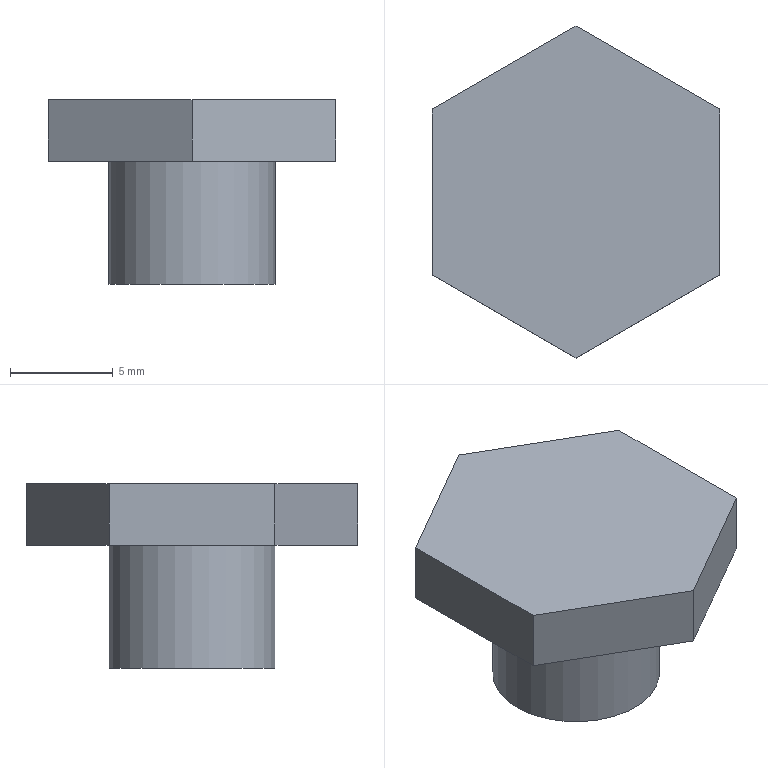Component | NX | PUNCH | 1 solid | 10 faces | box 14 x 16.17 x 9 mm | volume 818 mm3 | plane 9 | cylinder 1 | commonest cylinder face diameters 8.1 x1
STEP:
#1=CARTESIAN_POINT('',(0.,0.,0.));
#2=DIRECTION('',(0.,0.,1.));
#3=DIRECTION('',(1.,0.,0.));
#4=AXIS2_PLACEMENT_3D('',#1,#2,#3);
#5=CARTESIAN_POINT('',(-74.079,17.05,12.));
#6=VERTEX_POINT('',#5);
#7=CARTESIAN_POINT('',(-78.129,17.05,12.));
#8=DIRECTION('',(0.,0.,1.));
#9=DIRECTION('',(1.,0.,0.));
#10=AXIS2_PLACEMENT_3D('',#7,#8,#9);
#11=CIRCLE('',#10,4.05);
#12=CARTESIAN_POINT('',(-78.129,17.05,12.));
#13=DIRECTION('',(0.,0.,1.));
#14=DIRECTION('',(1.,0.,0.));
#15=AXIS2_PLACEMENT_3D('',#12,#13,#14);
#16=CYLINDRICAL_SURFACE('',#15,4.05);
#17=CARTESIAN_POINT('',(0.,0.));
#18=DIRECTION('',(1.,0.));
#19=VECTOR('',#18,1.);
#20=LINE('',#17,#19);
#21=(GEOMETRIC_REPRESENTATION_CONTEXT(2)PARAMETRIC_REPRESENTATION_CONTEXT()REPRESENTATION_CONTEXT('',''));
#22=DEFINITIONAL_REPRESENTATION('',(#20),#21);
#23=PCURVE('',#16,#22);
#24=CARTESIAN_POINT('',(-78.129,17.05,12.));
#25=DIRECTION('',(0.,0.,1.));
#26=DIRECTION('',(1.,0.,0.));
#27=AXIS2_PLACEMENT_3D('',#24,#25,#26);
#28=PLANE('',#27);
#29=CARTESIAN_POINT('',(0.,0.));
#30=DIRECTION('',(1.,0.));
#31=AXIS2_PLACEMENT_2D('',#29,#30);
#32=CIRCLE('',#31,4.05);
#33=(GEOMETRIC_REPRESENTATION_CONTEXT(2)PARAMETRIC_REPRESENTATION_CONTEXT()REPRESENTATION_CONTEXT('',''));
#34=DEFINITIONAL_REPRESENTATION('',(#32),#33);
#35=PCURVE('',#28,#34);
#36=SURFACE_CURVE('',#11,(#23,#35),.PCURVE_S1.);
#37=EDGE_CURVE('',#6,#6,#36,.T.);
#38=ORIENTED_EDGE('',*,*,#37,.T.);
#39=CARTESIAN_POINT('',(-74.079,17.05,18.));
#40=VERTEX_POINT('',#39);
#41=CARTESIAN_POINT('',(-74.079,17.05,12.));
#42=CARTESIAN_POINT('',(-74.079,17.05,18.));
#43=B_SPLINE_CURVE_WITH_KNOTS('',1,(#41,#42),.UNSPECIFIED.,.F.,.F.,(2,2),(0.,6.),.PIECEWISE_BEZIER_KNOTS.);
#44=CARTESIAN_POINT('',(6.283,0.));
#45=DIRECTION('',(0.,1.));
#46=VECTOR('',#45,1.);
#47=LINE('',#44,#46);
#48=(GEOMETRIC_REPRESENTATION_CONTEXT(2)PARAMETRIC_REPRESENTATION_CONTEXT()REPRESENTATION_CONTEXT('',''));
#49=DEFINITIONAL_REPRESENTATION('',(#47),#48);
#50=PCURVE('',#16,#49);
#51=CARTESIAN_POINT('',(0.,0.));
#52=DIRECTION('',(0.,1.));
#53=VECTOR('',#52,1.);
#54=LINE('',#51,#53);
#55=(GEOMETRIC_REPRESENTATION_CONTEXT(2)PARAMETRIC_REPRESENTATION_CONTEXT()REPRESENTATION_CONTEXT('',''));
#56=DEFINITIONAL_REPRESENTATION('',(#54),#55);
#57=PCURVE('',#16,#56);
#58=SEAM_CURVE('',#43,(#50,#57),.PCURVE_S1.);
#59=EDGE_CURVE('',#6,#40,#58,.T.);
#60=ORIENTED_EDGE('',*,*,#59,.T.);
#61=CARTESIAN_POINT('',(-78.129,17.05,18.));
#62=DIRECTION('',(0.,0.,1.));
#63=DIRECTION('',(1.,0.,0.));
#64=AXIS2_PLACEMENT_3D('',#61,#62,#63);
#65=CIRCLE('',#64,4.05);
#66=CARTESIAN_POINT('',(0.,6.));
#67=DIRECTION('',(1.,0.));
#68=VECTOR('',#67,1.);
#69=LINE('',#66,#68);
#70=(GEOMETRIC_REPRESENTATION_CONTEXT(2)PARAMETRIC_REPRESENTATION_CONTEXT()REPRESENTATION_CONTEXT('',''));
#71=DEFINITIONAL_REPRESENTATION('',(#69),#70);
#72=PCURVE('',#16,#71);
#73=CARTESIAN_POINT('',(-78.129,17.05,18.));
#74=DIRECTION('',(0.,0.,1.));
#75=DIRECTION('',(1.,0.,0.));
#76=AXIS2_PLACEMENT_3D('',#73,#74,#75);
#77=PLANE('',#76);
#78=CARTESIAN_POINT('',(0.,0.));
#79=DIRECTION('',(1.,0.));
#80=AXIS2_PLACEMENT_2D('',#78,#79);
#81=CIRCLE('',#80,4.05);
#82=(GEOMETRIC_REPRESENTATION_CONTEXT(2)PARAMETRIC_REPRESENTATION_CONTEXT()REPRESENTATION_CONTEXT('',''));
#83=DEFINITIONAL_REPRESENTATION('',(#81),#82);
#84=PCURVE('',#77,#83);
#85=SURFACE_CURVE('',#65,(#72,#84),.PCURVE_S1.);
#86=EDGE_CURVE('',#40,#40,#85,.T.);
#87=ORIENTED_EDGE('',*,*,#86,.F.);
#88=ORIENTED_EDGE('',*,*,#59,.F.);
#89=EDGE_LOOP('',(#38,#60,#87,#88));
#90=FACE_BOUND('',#89,.T.);
#91=ADVANCED_FACE('',(#90),#16,.T.);
#92=ORIENTED_EDGE('',*,*,#37,.F.);
#93=EDGE_LOOP('',(#92));
#94=FACE_BOUND('',#93,.T.);
#95=ADVANCED_FACE('',(#94),#28,.F.);
#96=CARTESIAN_POINT('',(-85.129,21.091,18.));
#97=VERTEX_POINT('',#96);
#98=CARTESIAN_POINT('',(-85.129,13.009,18.));
#99=VERTEX_POINT('',#98);
#100=CARTESIAN_POINT('',(-85.129,21.091,18.));
#101=DIRECTION('',(-0.,-1.,0.));
#102=VECTOR('',#101,1.);
#103=LINE('',#100,#102);
#104=CARTESIAN_POINT('',(-85.129,21.091,21.));
#105=DIRECTION('',(1.,-0.,0.));
#106=DIRECTION('',(0.,1.,0.));
#107=AXIS2_PLACEMENT_3D('',#104,#105,#106);
#108=PLANE('',#107);
#109=CARTESIAN_POINT('',(0.,-3.));
#110=DIRECTION('',(-1.,0.));
#111=VECTOR('',#110,1.);
#112=LINE('',#109,#111);
#113=(GEOMETRIC_REPRESENTATION_CONTEXT(2)PARAMETRIC_REPRESENTATION_CONTEXT()REPRESENTATION_CONTEXT('',''));
#114=DEFINITIONAL_REPRESENTATION('',(#112),#113);
#115=PCURVE('',#108,#114);
#116=CARTESIAN_POINT('',(-7.,4.041));
#117=DIRECTION('',(-0.,-1.));
#118=VECTOR('',#117,1.);
#119=LINE('',#116,#118);
#120=(GEOMETRIC_REPRESENTATION_CONTEXT(2)PARAMETRIC_REPRESENTATION_CONTEXT()REPRESENTATION_CONTEXT('',''));
#121=DEFINITIONAL_REPRESENTATION('',(#119),#120);
#122=PCURVE('',#77,#121);
#123=SURFACE_CURVE('',#103,(#115,#122),.PCURVE_S1.);
#124=EDGE_CURVE('',#97,#99,#123,.T.);
#125=ORIENTED_EDGE('',*,*,#124,.T.);
#126=CARTESIAN_POINT('',(-85.129,13.009,21.));
#127=VERTEX_POINT('',#126);
#128=CARTESIAN_POINT('',(-85.129,13.009,21.));
#129=DIRECTION('',(0.,0.,-1.));
#130=VECTOR('',#129,1.);
#131=LINE('',#128,#130);
#132=CARTESIAN_POINT('',(-8.083,0.));
#133=DIRECTION('',(0.,-1.));
#134=VECTOR('',#133,1.);
#135=LINE('',#132,#134);
#136=(GEOMETRIC_REPRESENTATION_CONTEXT(2)PARAMETRIC_REPRESENTATION_CONTEXT()REPRESENTATION_CONTEXT('',''));
#137=DEFINITIONAL_REPRESENTATION('',(#135),#136);
#138=PCURVE('',#108,#137);
#139=CARTESIAN_POINT('',(-85.129,13.009,21.));
#140=DIRECTION('',(0.5,0.866,0.));
#141=DIRECTION('',(-0.866,0.5,0.));
#142=AXIS2_PLACEMENT_3D('',#139,#140,#141);
#143=PLANE('',#142);
#144=CARTESIAN_POINT('',(0.,0.));
#145=DIRECTION('',(0.,-1.));
#146=VECTOR('',#145,1.);
#147=LINE('',#144,#146);
#148=(GEOMETRIC_REPRESENTATION_CONTEXT(2)PARAMETRIC_REPRESENTATION_CONTEXT()REPRESENTATION_CONTEXT('',''));
#149=DEFINITIONAL_REPRESENTATION('',(#147),#148);
#150=PCURVE('',#143,#149);
#151=SURFACE_CURVE('',#131,(#138,#150),.PCURVE_S1.);
#152=EDGE_CURVE('',#127,#99,#151,.T.);
#153=ORIENTED_EDGE('',*,*,#152,.F.);
#154=CARTESIAN_POINT('',(-85.129,21.091,21.));
#155=VERTEX_POINT('',#154);
#156=CARTESIAN_POINT('',(-85.129,21.091,21.));
#157=DIRECTION('',(-0.,-1.,0.));
#158=VECTOR('',#157,1.);
#159=LINE('',#156,#158);
#160=CARTESIAN_POINT('',(0.,0.));
#161=DIRECTION('',(-1.,0.));
#162=VECTOR('',#161,1.);
#163=LINE('',#160,#162);
#164=(GEOMETRIC_REPRESENTATION_CONTEXT(2)PARAMETRIC_REPRESENTATION_CONTEXT()REPRESENTATION_CONTEXT('',''));
#165=DEFINITIONAL_REPRESENTATION('',(#163),#164);
#166=PCURVE('',#108,#165);
#167=CARTESIAN_POINT('',(-78.129,17.05,21.));
#168=DIRECTION('',(0.,0.,1.));
#169=DIRECTION('',(1.,0.,0.));
#170=AXIS2_PLACEMENT_3D('',#167,#168,#169);
#171=PLANE('',#170);
#172=CARTESIAN_POINT('',(-7.,4.041));
#173=DIRECTION('',(-0.,-1.));
#174=VECTOR('',#173,1.);
#175=LINE('',#172,#174);
#176=(GEOMETRIC_REPRESENTATION_CONTEXT(2)PARAMETRIC_REPRESENTATION_CONTEXT()REPRESENTATION_CONTEXT('',''));
#177=DEFINITIONAL_REPRESENTATION('',(#175),#176);
#178=PCURVE('',#171,#177);
#179=SURFACE_CURVE('',#159,(#166,#178),.PCURVE_S1.);
#180=EDGE_CURVE('',#155,#127,#179,.T.);
#181=ORIENTED_EDGE('',*,*,#180,.F.);
#182=CARTESIAN_POINT('',(-85.129,21.091,21.));
#183=DIRECTION('',(0.,0.,-1.));
#184=VECTOR('',#183,1.);
#185=LINE('',#182,#184);
#186=CARTESIAN_POINT('',(0.,0.));
#187=DIRECTION('',(0.,-1.));
#188=VECTOR('',#187,1.);
#189=LINE('',#186,#188);
#190=(GEOMETRIC_REPRESENTATION_CONTEXT(2)PARAMETRIC_REPRESENTATION_CONTEXT()REPRESENTATION_CONTEXT('',''));
#191=DEFINITIONAL_REPRESENTATION('',(#189),#190);
#192=PCURVE('',#108,#191);
#193=CARTESIAN_POINT('',(-78.129,25.133,21.));
#194=DIRECTION('',(0.5,-0.866,0.));
#195=DIRECTION('',(0.866,0.5,0.));
#196=AXIS2_PLACEMENT_3D('',#193,#194,#195);
#197=PLANE('',#196);
#198=CARTESIAN_POINT('',(-8.083,0.));
#199=DIRECTION('',(0.,-1.));
#200=VECTOR('',#199,1.);
#201=LINE('',#198,#200);
#202=(GEOMETRIC_REPRESENTATION_CONTEXT(2)PARAMETRIC_REPRESENTATION_CONTEXT()REPRESENTATION_CONTEXT('',''));
#203=DEFINITIONAL_REPRESENTATION('',(#201),#202);
#204=PCURVE('',#197,#203);
#205=SURFACE_CURVE('',#185,(#192,#204),.PCURVE_S1.);
#206=EDGE_CURVE('',#155,#97,#205,.T.);
#207=ORIENTED_EDGE('',*,*,#206,.T.);
#208=EDGE_LOOP('',(#125,#153,#181,#207));
#209=FACE_BOUND('',#208,.T.);
#210=ADVANCED_FACE('',(#209),#108,.F.);
#211=CARTESIAN_POINT('',(-78.129,8.967,18.));
#212=VERTEX_POINT('',#211);
#213=CARTESIAN_POINT('',(-85.129,13.009,18.));
#214=DIRECTION('',(0.866,-0.5,0.));
#215=VECTOR('',#214,1.);
#216=LINE('',#213,#215);
#217=CARTESIAN_POINT('',(0.,-3.));
#218=DIRECTION('',(-1.,0.));
#219=VECTOR('',#218,1.);
#220=LINE('',#217,#219);
#221=(GEOMETRIC_REPRESENTATION_CONTEXT(2)PARAMETRIC_REPRESENTATION_CONTEXT()REPRESENTATION_CONTEXT('',''));
#222=DEFINITIONAL_REPRESENTATION('',(#220),#221);
#223=PCURVE('',#143,#222);
#224=CARTESIAN_POINT('',(-7.,-4.041));
#225=DIRECTION('',(0.866,-0.5));
#226=VECTOR('',#225,1.);
#227=LINE('',#224,#226);
#228=(GEOMETRIC_REPRESENTATION_CONTEXT(2)PARAMETRIC_REPRESENTATION_CONTEXT()REPRESENTATION_CONTEXT('',''));
#229=DEFINITIONAL_REPRESENTATION('',(#227),#228);
#230=PCURVE('',#77,#229);
#231=SURFACE_CURVE('',#216,(#223,#230),.PCURVE_S1.);
#232=EDGE_CURVE('',#99,#212,#231,.T.);
#233=ORIENTED_EDGE('',*,*,#232,.T.);
#234=CARTESIAN_POINT('',(-78.129,8.967,21.));
#235=VERTEX_POINT('',#234);
#236=CARTESIAN_POINT('',(-78.129,8.967,21.));
#237=DIRECTION('',(0.,0.,-1.));
#238=VECTOR('',#237,1.);
#239=LINE('',#236,#238);
#240=CARTESIAN_POINT('',(-8.083,0.));
#241=DIRECTION('',(0.,-1.));
#242=VECTOR('',#241,1.);
#243=LINE('',#240,#242);
#244=(GEOMETRIC_REPRESENTATION_CONTEXT(2)PARAMETRIC_REPRESENTATION_CONTEXT()REPRESENTATION_CONTEXT('',''));
#245=DEFINITIONAL_REPRESENTATION('',(#243),#244);
#246=PCURVE('',#143,#245);
#247=CARTESIAN_POINT('',(-78.129,8.967,21.));
#248=DIRECTION('',(-0.5,0.866,0.));
#249=DIRECTION('',(-0.866,-0.5,0.));
#250=AXIS2_PLACEMENT_3D('',#247,#248,#249);
#251=PLANE('',#250);
#252=CARTESIAN_POINT('',(-0.,0.));
#253=DIRECTION('',(0.,-1.));
#254=VECTOR('',#253,1.);
#255=LINE('',#252,#254);
#256=(GEOMETRIC_REPRESENTATION_CONTEXT(2)PARAMETRIC_REPRESENTATION_CONTEXT()REPRESENTATION_CONTEXT('',''));
#257=DEFINITIONAL_REPRESENTATION('',(#255),#256);
#258=PCURVE('',#251,#257);
#259=SURFACE_CURVE('',#239,(#246,#258),.PCURVE_S1.);
#260=EDGE_CURVE('',#235,#212,#259,.T.);
#261=ORIENTED_EDGE('',*,*,#260,.F.);
#262=CARTESIAN_POINT('',(-85.129,13.009,21.));
#263=DIRECTION('',(0.866,-0.5,0.));
#264=VECTOR('',#263,1.);
#265=LINE('',#262,#264);
#266=CARTESIAN_POINT('',(0.,0.));
#267=DIRECTION('',(-1.,0.));
#268=VECTOR('',#267,1.);
#269=LINE('',#266,#268);
#270=(GEOMETRIC_REPRESENTATION_CONTEXT(2)PARAMETRIC_REPRESENTATION_CONTEXT()REPRESENTATION_CONTEXT('',''));
#271=DEFINITIONAL_REPRESENTATION('',(#269),#270);
#272=PCURVE('',#143,#271);
#273=CARTESIAN_POINT('',(-7.,-4.041));
#274=DIRECTION('',(0.866,-0.5));
#275=VECTOR('',#274,1.);
#276=LINE('',#273,#275);
#277=(GEOMETRIC_REPRESENTATION_CONTEXT(2)PARAMETRIC_REPRESENTATION_CONTEXT()REPRESENTATION_CONTEXT('',''));
#278=DEFINITIONAL_REPRESENTATION('',(#276),#277);
#279=PCURVE('',#171,#278);
#280=SURFACE_CURVE('',#265,(#272,#279),.PCURVE_S1.);
#281=EDGE_CURVE('',#127,#235,#280,.T.);
#282=ORIENTED_EDGE('',*,*,#281,.F.);
#283=ORIENTED_EDGE('',*,*,#152,.T.);
#284=EDGE_LOOP('',(#233,#261,#282,#283));
#285=FACE_BOUND('',#284,.T.);
#286=ADVANCED_FACE('',(#285),#143,.F.);
#287=CARTESIAN_POINT('',(-71.129,13.009,18.));
#288=VERTEX_POINT('',#287);
#289=CARTESIAN_POINT('',(-78.129,8.967,18.));
#290=DIRECTION('',(0.866,0.5,0.));
#291=VECTOR('',#290,1.);
#292=LINE('',#289,#291);
#293=CARTESIAN_POINT('',(0.,-3.));
#294=DIRECTION('',(-1.,0.));
#295=VECTOR('',#294,1.);
#296=LINE('',#293,#295);
#297=(GEOMETRIC_REPRESENTATION_CONTEXT(2)PARAMETRIC_REPRESENTATION_CONTEXT()REPRESENTATION_CONTEXT('',''));
#298=DEFINITIONAL_REPRESENTATION('',(#296),#297);
#299=PCURVE('',#251,#298);
#300=CARTESIAN_POINT('',(0.,-8.083));
#301=DIRECTION('',(0.866,0.5));
#302=VECTOR('',#301,1.);
#303=LINE('',#300,#302);
#304=(GEOMETRIC_REPRESENTATION_CONTEXT(2)PARAMETRIC_REPRESENTATION_CONTEXT()REPRESENTATION_CONTEXT('',''));
#305=DEFINITIONAL_REPRESENTATION('',(#303),#304);
#306=PCURVE('',#77,#305);
#307=SURFACE_CURVE('',#292,(#299,#306),.PCURVE_S1.);
#308=EDGE_CURVE('',#212,#288,#307,.T.);
#309=ORIENTED_EDGE('',*,*,#308,.T.);
#310=CARTESIAN_POINT('',(-71.129,13.009,21.));
#311=VERTEX_POINT('',#310);
#312=CARTESIAN_POINT('',(-71.129,13.009,21.));
#313=DIRECTION('',(0.,0.,-1.));
#314=VECTOR('',#313,1.);
#315=LINE('',#312,#314);
#316=CARTESIAN_POINT('',(-8.083,0.));
#317=DIRECTION('',(0.,-1.));
#318=VECTOR('',#317,1.);
#319=LINE('',#316,#318);
#320=(GEOMETRIC_REPRESENTATION_CONTEXT(2)PARAMETRIC_REPRESENTATION_CONTEXT()REPRESENTATION_CONTEXT('',''));
#321=DEFINITIONAL_REPRESENTATION('',(#319),#320);
#322=PCURVE('',#251,#321);
#323=CARTESIAN_POINT('',(-71.129,13.009,21.));
#324=DIRECTION('',(-1.,-0.,0.));
#325=DIRECTION('',(0.,-1.,0.));
#326=AXIS2_PLACEMENT_3D('',#323,#324,#325);
#327=PLANE('',#326);
#328=CARTESIAN_POINT('',(0.,0.));
#329=DIRECTION('',(0.,-1.));
#330=VECTOR('',#329,1.);
#331=LINE('',#328,#330);
#332=(GEOMETRIC_REPRESENTATION_CONTEXT(2)PARAMETRIC_REPRESENTATION_CONTEXT()REPRESENTATION_CONTEXT('',''));
#333=DEFINITIONAL_REPRESENTATION('',(#331),#332);
#334=PCURVE('',#327,#333);
#335=SURFACE_CURVE('',#315,(#322,#334),.PCURVE_S1.);
#336=EDGE_CURVE('',#311,#288,#335,.T.);
#337=ORIENTED_EDGE('',*,*,#336,.F.);
#338=CARTESIAN_POINT('',(-78.129,8.967,21.));
#339=DIRECTION('',(0.866,0.5,0.));
#340=VECTOR('',#339,1.);
#341=LINE('',#338,#340);
#342=CARTESIAN_POINT('',(0.,0.));
#343=DIRECTION('',(-1.,0.));
#344=VECTOR('',#343,1.);
#345=LINE('',#342,#344);
#346=(GEOMETRIC_REPRESENTATION_CONTEXT(2)PARAMETRIC_REPRESENTATION_CONTEXT()REPRESENTATION_CONTEXT('',''));
#347=DEFINITIONAL_REPRESENTATION('',(#345),#346);
#348=PCURVE('',#251,#347);
#349=CARTESIAN_POINT('',(0.,-8.083));
#350=DIRECTION('',(0.866,0.5));
#351=VECTOR('',#350,1.);
#352=LINE('',#349,#351);
#353=(GEOMETRIC_REPRESENTATION_CONTEXT(2)PARAMETRIC_REPRESENTATION_CONTEXT()REPRESENTATION_CONTEXT('',''));
#354=DEFINITIONAL_REPRESENTATION('',(#352),#353);
#355=PCURVE('',#171,#354);
#356=SURFACE_CURVE('',#341,(#348,#355),.PCURVE_S1.);
#357=EDGE_CURVE('',#235,#311,#356,.T.);
#358=ORIENTED_EDGE('',*,*,#357,.F.);
#359=ORIENTED_EDGE('',*,*,#260,.T.);
#360=EDGE_LOOP('',(#309,#337,#358,#359));
#361=FACE_BOUND('',#360,.T.);
#362=ADVANCED_FACE('',(#361),#251,.F.);
#363=CARTESIAN_POINT('',(-71.129,21.091,18.));
#364=VERTEX_POINT('',#363);
#365=CARTESIAN_POINT('',(-71.129,13.009,18.));
#366=DIRECTION('',(-0.,1.,0.));
#367=VECTOR('',#366,1.);
#368=LINE('',#365,#367);
#369=CARTESIAN_POINT('',(0.,-3.));
#370=DIRECTION('',(-1.,0.));
#371=VECTOR('',#370,1.);
#372=LINE('',#369,#371);
#373=(GEOMETRIC_REPRESENTATION_CONTEXT(2)PARAMETRIC_REPRESENTATION_CONTEXT()REPRESENTATION_CONTEXT('',''));
#374=DEFINITIONAL_REPRESENTATION('',(#372),#373);
#375=PCURVE('',#327,#374);
#376=CARTESIAN_POINT('',(7.,-4.041));
#377=DIRECTION('',(-0.,1.));
#378=VECTOR('',#377,1.);
#379=LINE('',#376,#378);
#380=(GEOMETRIC_REPRESENTATION_CONTEXT(2)PARAMETRIC_REPRESENTATION_CONTEXT()REPRESENTATION_CONTEXT('',''));
#381=DEFINITIONAL_REPRESENTATION('',(#379),#380);
#382=PCURVE('',#77,#381);
#383=SURFACE_CURVE('',#368,(#375,#382),.PCURVE_S1.);
#384=EDGE_CURVE('',#288,#364,#383,.T.);
#385=ORIENTED_EDGE('',*,*,#384,.T.);
#386=CARTESIAN_POINT('',(-71.129,21.091,21.));
#387=VERTEX_POINT('',#386);
#388=CARTESIAN_POINT('',(-71.129,21.091,21.));
#389=DIRECTION('',(0.,0.,-1.));
#390=VECTOR('',#389,1.);
#391=LINE('',#388,#390);
#392=CARTESIAN_POINT('',(-8.083,0.));
#393=DIRECTION('',(0.,-1.));
#394=VECTOR('',#393,1.);
#395=LINE('',#392,#394);
#396=(GEOMETRIC_REPRESENTATION_CONTEXT(2)PARAMETRIC_REPRESENTATION_CONTEXT()REPRESENTATION_CONTEXT('',''));
#397=DEFINITIONAL_REPRESENTATION('',(#395),#396);
#398=PCURVE('',#327,#397);
#399=CARTESIAN_POINT('',(-71.129,21.091,21.));
#400=DIRECTION('',(-0.5,-0.866,0.));
#401=DIRECTION('',(0.866,-0.5,0.));
#402=AXIS2_PLACEMENT_3D('',#399,#400,#401);
#403=PLANE('',#402);
#404=CARTESIAN_POINT('',(0.,0.));
#405=DIRECTION('',(0.,-1.));
#406=VECTOR('',#405,1.);
#407=LINE('',#404,#406);
#408=(GEOMETRIC_REPRESENTATION_CONTEXT(2)PARAMETRIC_REPRESENTATION_CONTEXT()REPRESENTATION_CONTEXT('',''));
#409=DEFINITIONAL_REPRESENTATION('',(#407),#408);
#410=PCURVE('',#403,#409);
#411=SURFACE_CURVE('',#391,(#398,#410),.PCURVE_S1.);
#412=EDGE_CURVE('',#387,#364,#411,.T.);
#413=ORIENTED_EDGE('',*,*,#412,.F.);
#414=CARTESIAN_POINT('',(-71.129,13.009,21.));
#415=DIRECTION('',(-0.,1.,0.));
#416=VECTOR('',#415,1.);
#417=LINE('',#414,#416);
#418=CARTESIAN_POINT('',(0.,0.));
#419=DIRECTION('',(-1.,0.));
#420=VECTOR('',#419,1.);
#421=LINE('',#418,#420);
#422=(GEOMETRIC_REPRESENTATION_CONTEXT(2)PARAMETRIC_REPRESENTATION_CONTEXT()REPRESENTATION_CONTEXT('',''));
#423=DEFINITIONAL_REPRESENTATION('',(#421),#422);
#424=PCURVE('',#327,#423);
#425=CARTESIAN_POINT('',(7.,-4.041));
#426=DIRECTION('',(-0.,1.));
#427=VECTOR('',#426,1.);
#428=LINE('',#425,#427);
#429=(GEOMETRIC_REPRESENTATION_CONTEXT(2)PARAMETRIC_REPRESENTATION_CONTEXT()REPRESENTATION_CONTEXT('',''));
#430=DEFINITIONAL_REPRESENTATION('',(#428),#429);
#431=PCURVE('',#171,#430);
#432=SURFACE_CURVE('',#417,(#424,#431),.PCURVE_S1.);
#433=EDGE_CURVE('',#311,#387,#432,.T.);
#434=ORIENTED_EDGE('',*,*,#433,.F.);
#435=ORIENTED_EDGE('',*,*,#336,.T.);
#436=EDGE_LOOP('',(#385,#413,#434,#435));
#437=FACE_BOUND('',#436,.T.);
#438=ADVANCED_FACE('',(#437),#327,.F.);
#439=CARTESIAN_POINT('',(-78.129,25.133,18.));
#440=VERTEX_POINT('',#439);
#441=CARTESIAN_POINT('',(-71.129,21.091,18.));
#442=DIRECTION('',(-0.866,0.5,0.));
#443=VECTOR('',#442,1.);
#444=LINE('',#441,#443);
#445=CARTESIAN_POINT('',(0.,-3.));
#446=DIRECTION('',(-1.,0.));
#447=VECTOR('',#446,1.);
#448=LINE('',#445,#447);
#449=(GEOMETRIC_REPRESENTATION_CONTEXT(2)PARAMETRIC_REPRESENTATION_CONTEXT()REPRESENTATION_CONTEXT('',''));
#450=DEFINITIONAL_REPRESENTATION('',(#448),#449);
#451=PCURVE('',#403,#450);
#452=CARTESIAN_POINT('',(7.,4.041));
#453=DIRECTION('',(-0.866,0.5));
#454=VECTOR('',#453,1.);
#455=LINE('',#452,#454);
#456=(GEOMETRIC_REPRESENTATION_CONTEXT(2)PARAMETRIC_REPRESENTATION_CONTEXT()REPRESENTATION_CONTEXT('',''));
#457=DEFINITIONAL_REPRESENTATION('',(#455),#456);
#458=PCURVE('',#77,#457);
#459=SURFACE_CURVE('',#444,(#451,#458),.PCURVE_S1.);
#460=EDGE_CURVE('',#364,#440,#459,.T.);
#461=ORIENTED_EDGE('',*,*,#460,.T.);
#462=CARTESIAN_POINT('',(-78.129,25.133,21.));
#463=VERTEX_POINT('',#462);
#464=CARTESIAN_POINT('',(-78.129,25.133,21.));
#465=DIRECTION('',(0.,0.,-1.));
#466=VECTOR('',#465,1.);
#467=LINE('',#464,#466);
#468=CARTESIAN_POINT('',(-8.083,0.));
#469=DIRECTION('',(0.,-1.));
#470=VECTOR('',#469,1.);
#471=LINE('',#468,#470);
#472=(GEOMETRIC_REPRESENTATION_CONTEXT(2)PARAMETRIC_REPRESENTATION_CONTEXT()REPRESENTATION_CONTEXT('',''));
#473=DEFINITIONAL_REPRESENTATION('',(#471),#472);
#474=PCURVE('',#403,#473);
#475=CARTESIAN_POINT('',(0.,0.));
#476=DIRECTION('',(0.,-1.));
#477=VECTOR('',#476,1.);
#478=LINE('',#475,#477);
#479=(GEOMETRIC_REPRESENTATION_CONTEXT(2)PARAMETRIC_REPRESENTATION_CONTEXT()REPRESENTATION_CONTEXT('',''));
#480=DEFINITIONAL_REPRESENTATION('',(#478),#479);
#481=PCURVE('',#197,#480);
#482=SURFACE_CURVE('',#467,(#474,#481),.PCURVE_S1.);
#483=EDGE_CURVE('',#463,#440,#482,.T.);
#484=ORIENTED_EDGE('',*,*,#483,.F.);
#485=CARTESIAN_POINT('',(-71.129,21.091,21.));
#486=DIRECTION('',(-0.866,0.5,0.));
#487=VECTOR('',#486,1.);
#488=LINE('',#485,#487);
#489=CARTESIAN_POINT('',(0.,0.));
#490=DIRECTION('',(-1.,0.));
#491=VECTOR('',#490,1.);
#492=LINE('',#489,#491);
#493=(GEOMETRIC_REPRESENTATION_CONTEXT(2)PARAMETRIC_REPRESENTATION_CONTEXT()REPRESENTATION_CONTEXT('',''));
#494=DEFINITIONAL_REPRESENTATION('',(#492),#493);
#495=PCURVE('',#403,#494);
#496=CARTESIAN_POINT('',(7.,4.041));
#497=DIRECTION('',(-0.866,0.5));
#498=VECTOR('',#497,1.);
#499=LINE('',#496,#498);
#500=(GEOMETRIC_REPRESENTATION_CONTEXT(2)PARAMETRIC_REPRESENTATION_CONTEXT()REPRESENTATION_CONTEXT('',''));
#501=DEFINITIONAL_REPRESENTATION('',(#499),#500);
#502=PCURVE('',#171,#501);
#503=SURFACE_CURVE('',#488,(#495,#502),.PCURVE_S1.);
#504=EDGE_CURVE('',#387,#463,#503,.T.);
#505=ORIENTED_EDGE('',*,*,#504,.F.);
#506=ORIENTED_EDGE('',*,*,#412,.T.);
#507=EDGE_LOOP('',(#461,#484,#505,#506));
#508=FACE_BOUND('',#507,.T.);
#509=ADVANCED_FACE('',(#508),#403,.F.);
#510=CARTESIAN_POINT('',(-78.129,25.133,18.));
#511=DIRECTION('',(-0.866,-0.5,0.));
#512=VECTOR('',#511,1.);
#513=LINE('',#510,#512);
#514=CARTESIAN_POINT('',(0.,-3.));
#515=DIRECTION('',(-1.,0.));
#516=VECTOR('',#515,1.);
#517=LINE('',#514,#516);
#518=(GEOMETRIC_REPRESENTATION_CONTEXT(2)PARAMETRIC_REPRESENTATION_CONTEXT()REPRESENTATION_CONTEXT('',''));
#519=DEFINITIONAL_REPRESENTATION('',(#517),#518);
#520=PCURVE('',#197,#519);
#521=CARTESIAN_POINT('',(0.,8.083));
#522=DIRECTION('',(-0.866,-0.5));
#523=VECTOR('',#522,1.);
#524=LINE('',#521,#523);
#525=(GEOMETRIC_REPRESENTATION_CONTEXT(2)PARAMETRIC_REPRESENTATION_CONTEXT()REPRESENTATION_CONTEXT('',''));
#526=DEFINITIONAL_REPRESENTATION('',(#524),#525);
#527=PCURVE('',#77,#526);
#528=SURFACE_CURVE('',#513,(#520,#527),.PCURVE_S1.);
#529=EDGE_CURVE('',#440,#97,#528,.T.);
#530=ORIENTED_EDGE('',*,*,#529,.T.);
#531=ORIENTED_EDGE('',*,*,#206,.F.);
#532=CARTESIAN_POINT('',(-78.129,25.133,21.));
#533=DIRECTION('',(-0.866,-0.5,0.));
#534=VECTOR('',#533,1.);
#535=LINE('',#532,#534);
#536=CARTESIAN_POINT('',(0.,0.));
#537=DIRECTION('',(-1.,0.));
#538=VECTOR('',#537,1.);
#539=LINE('',#536,#538);
#540=(GEOMETRIC_REPRESENTATION_CONTEXT(2)PARAMETRIC_REPRESENTATION_CONTEXT()REPRESENTATION_CONTEXT('',''));
#541=DEFINITIONAL_REPRESENTATION('',(#539),#540);
#542=PCURVE('',#197,#541);
#543=CARTESIAN_POINT('',(0.,8.083));
#544=DIRECTION('',(-0.866,-0.5));
#545=VECTOR('',#544,1.);
#546=LINE('',#543,#545);
#547=(GEOMETRIC_REPRESENTATION_CONTEXT(2)PARAMETRIC_REPRESENTATION_CONTEXT()REPRESENTATION_CONTEXT('',''));
#548=DEFINITIONAL_REPRESENTATION('',(#546),#547);
#549=PCURVE('',#171,#548);
#550=SURFACE_CURVE('',#535,(#542,#549),.PCURVE_S1.);
#551=EDGE_CURVE('',#463,#155,#550,.T.);
#552=ORIENTED_EDGE('',*,*,#551,.F.);
#553=ORIENTED_EDGE('',*,*,#483,.T.);
#554=EDGE_LOOP('',(#530,#531,#552,#553));
#555=FACE_BOUND('',#554,.T.);
#556=ADVANCED_FACE('',(#555),#197,.F.);
#557=ORIENTED_EDGE('',*,*,#124,.F.);
#558=ORIENTED_EDGE('',*,*,#529,.F.);
#559=ORIENTED_EDGE('',*,*,#460,.F.);
#560=ORIENTED_EDGE('',*,*,#384,.F.);
#561=ORIENTED_EDGE('',*,*,#308,.F.);
#562=ORIENTED_EDGE('',*,*,#232,.F.);
#563=EDGE_LOOP('',(#557,#558,#559,#560,#561,#562));
#564=FACE_BOUND('',#563,.T.);
#565=ORIENTED_EDGE('',*,*,#86,.T.);
#566=EDGE_LOOP('',(#565));
#567=FACE_BOUND('',#566,.T.);
#568=ADVANCED_FACE('',(#564,#567),#77,.F.);
#569=ORIENTED_EDGE('',*,*,#180,.T.);
#570=ORIENTED_EDGE('',*,*,#281,.T.);
#571=ORIENTED_EDGE('',*,*,#357,.T.);
#572=ORIENTED_EDGE('',*,*,#433,.T.);
#573=ORIENTED_EDGE('',*,*,#504,.T.);
#574=ORIENTED_EDGE('',*,*,#551,.T.);
#575=EDGE_LOOP('',(#569,#570,#571,#572,#573,#574));
#576=FACE_BOUND('',#575,.T.);
#577=ADVANCED_FACE('',(#576),#171,.T.);
#578=CLOSED_SHELL('',(#91,#95,#210,#286,#362,#438,#509,#556,#568,#577));
#579=MANIFOLD_SOLID_BREP('',#578);
#580=(LENGTH_UNIT()NAMED_UNIT(*)SI_UNIT(.MILLI.,.METRE.));
#581=UNCERTAINTY_MEASURE_WITH_UNIT(LENGTH_MEASURE(0.000001),#580,'','');
#582=(NAMED_UNIT(*)PLANE_ANGLE_UNIT()SI_UNIT($,.RADIAN.));
#583=(NAMED_UNIT(*)SI_UNIT($,.STERADIAN.)SOLID_ANGLE_UNIT());
#584=(GEOMETRIC_REPRESENTATION_CONTEXT(3)GLOBAL_UNCERTAINTY_ASSIGNED_CONTEXT((#581))GLOBAL_UNIT_ASSIGNED_CONTEXT((#580,#582,#583))REPRESENTATION_CONTEXT('',''));
#585=ADVANCED_BREP_SHAPE_REPRESENTATION('',(#4,#579),#584);